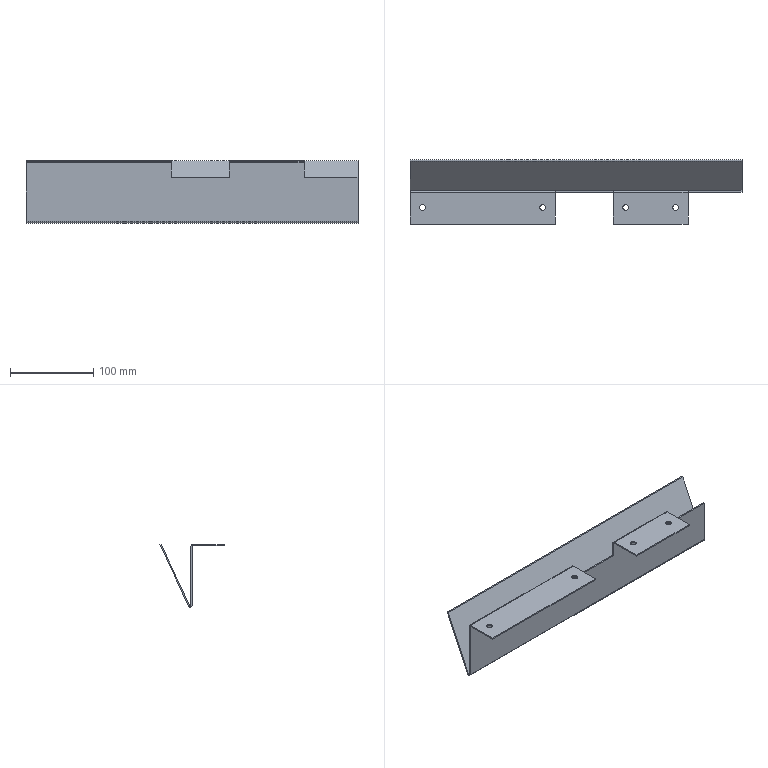Component | SolidWorks | Q1-A12-S21-Q4-08B-2 | 1 solid | 44 faces | volume 105888 mm3 | plane 30 | cylinder 14 | commonest cylinder face diameters 7 x8 4.473 x3 1.473 x3 | material SUS-304